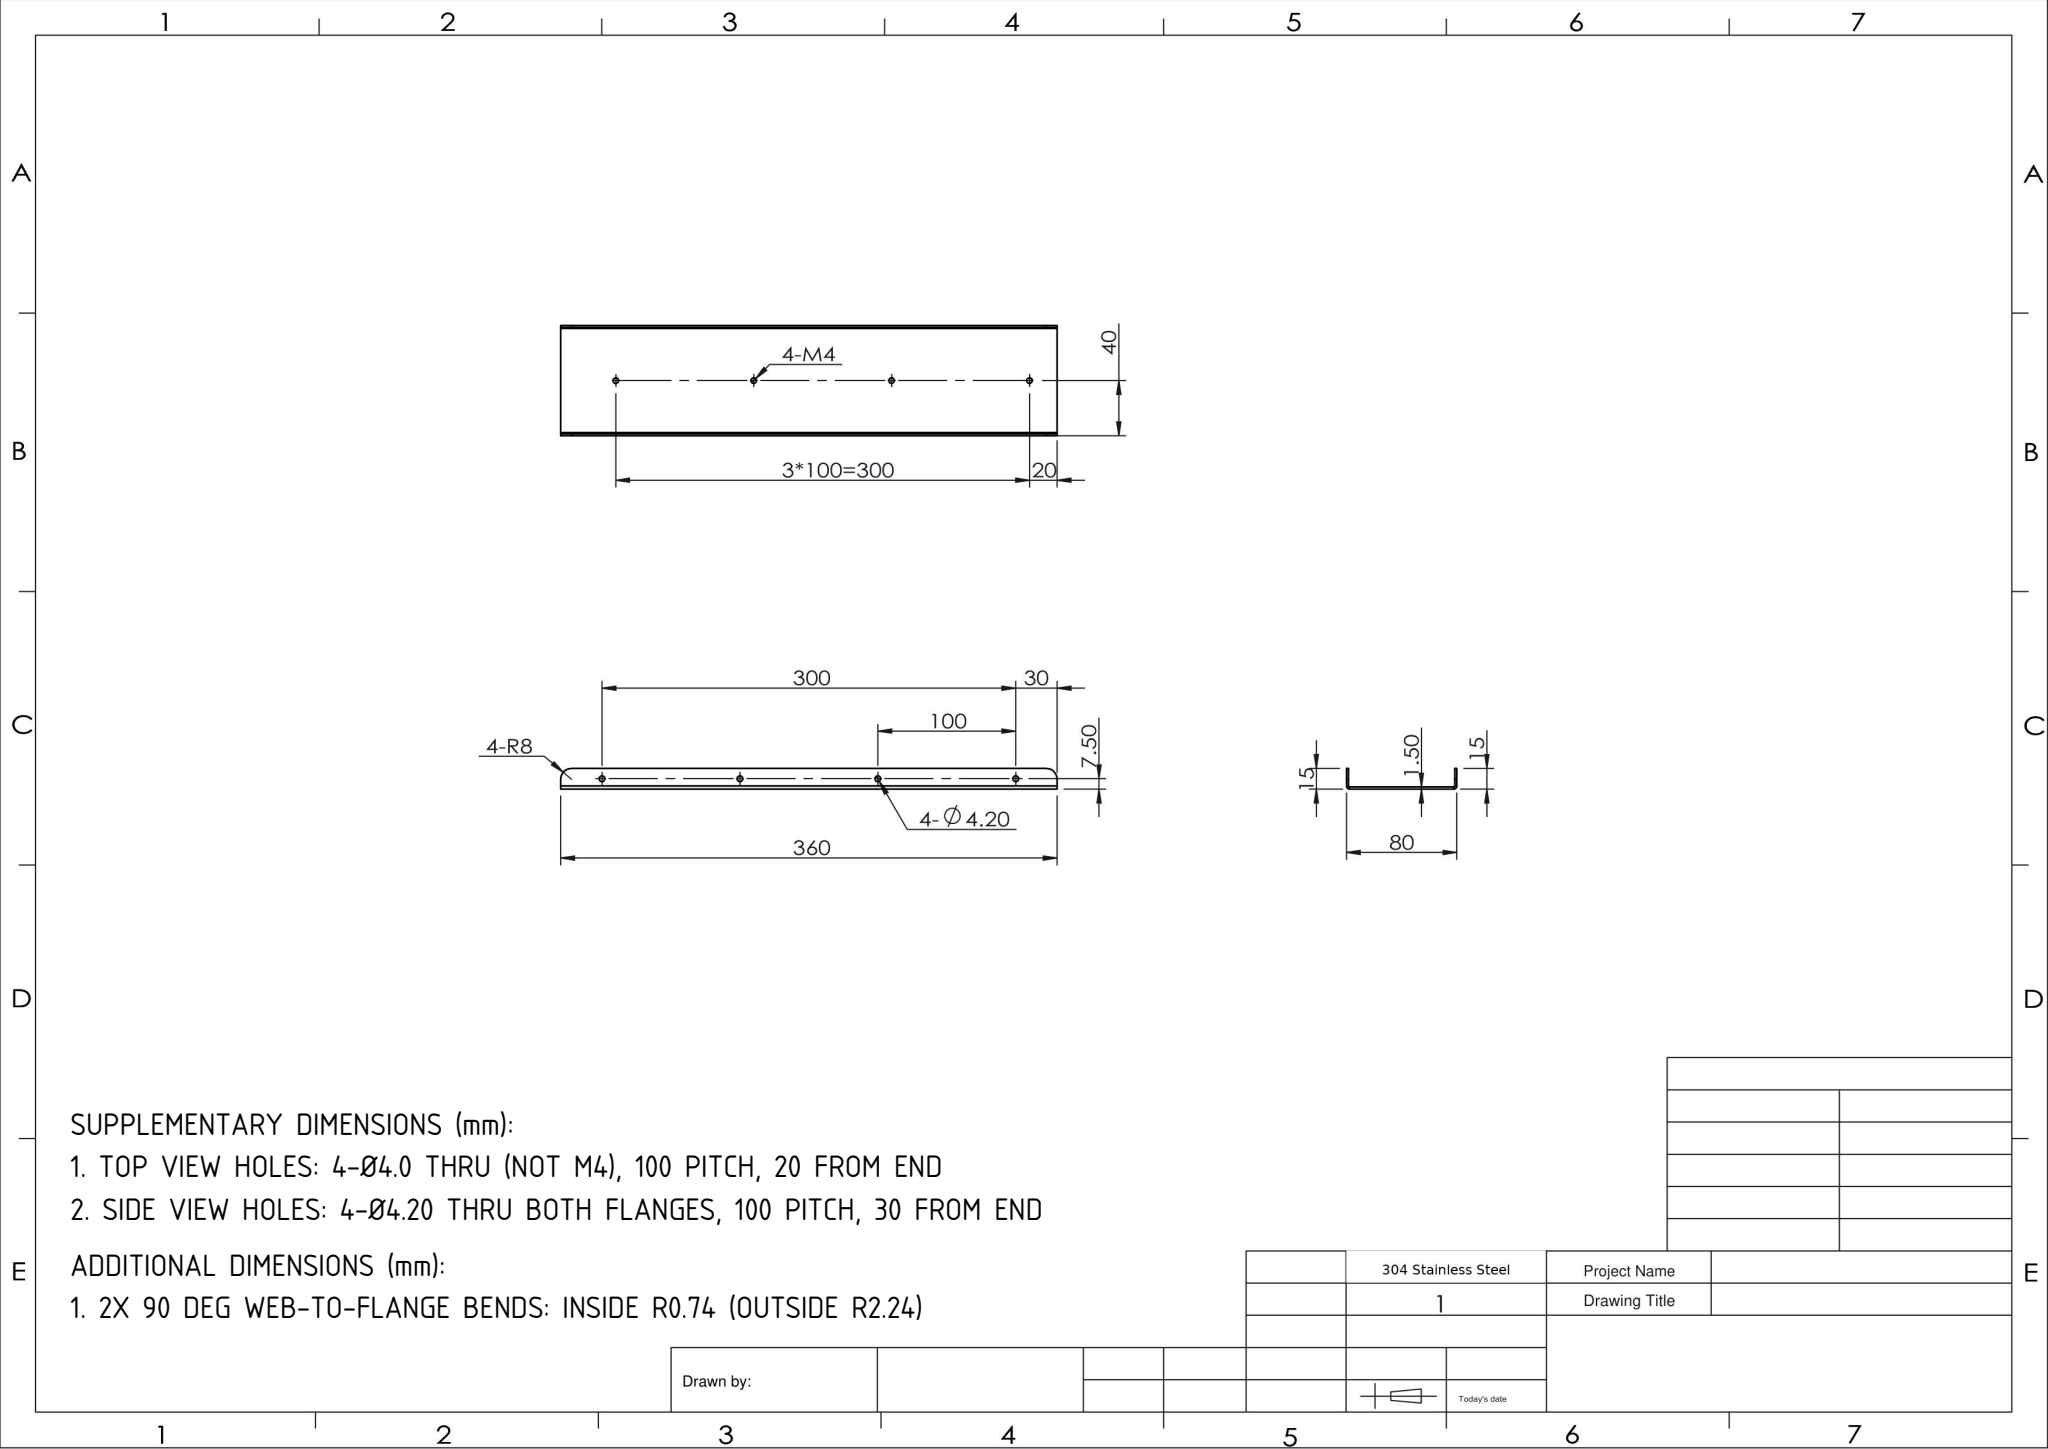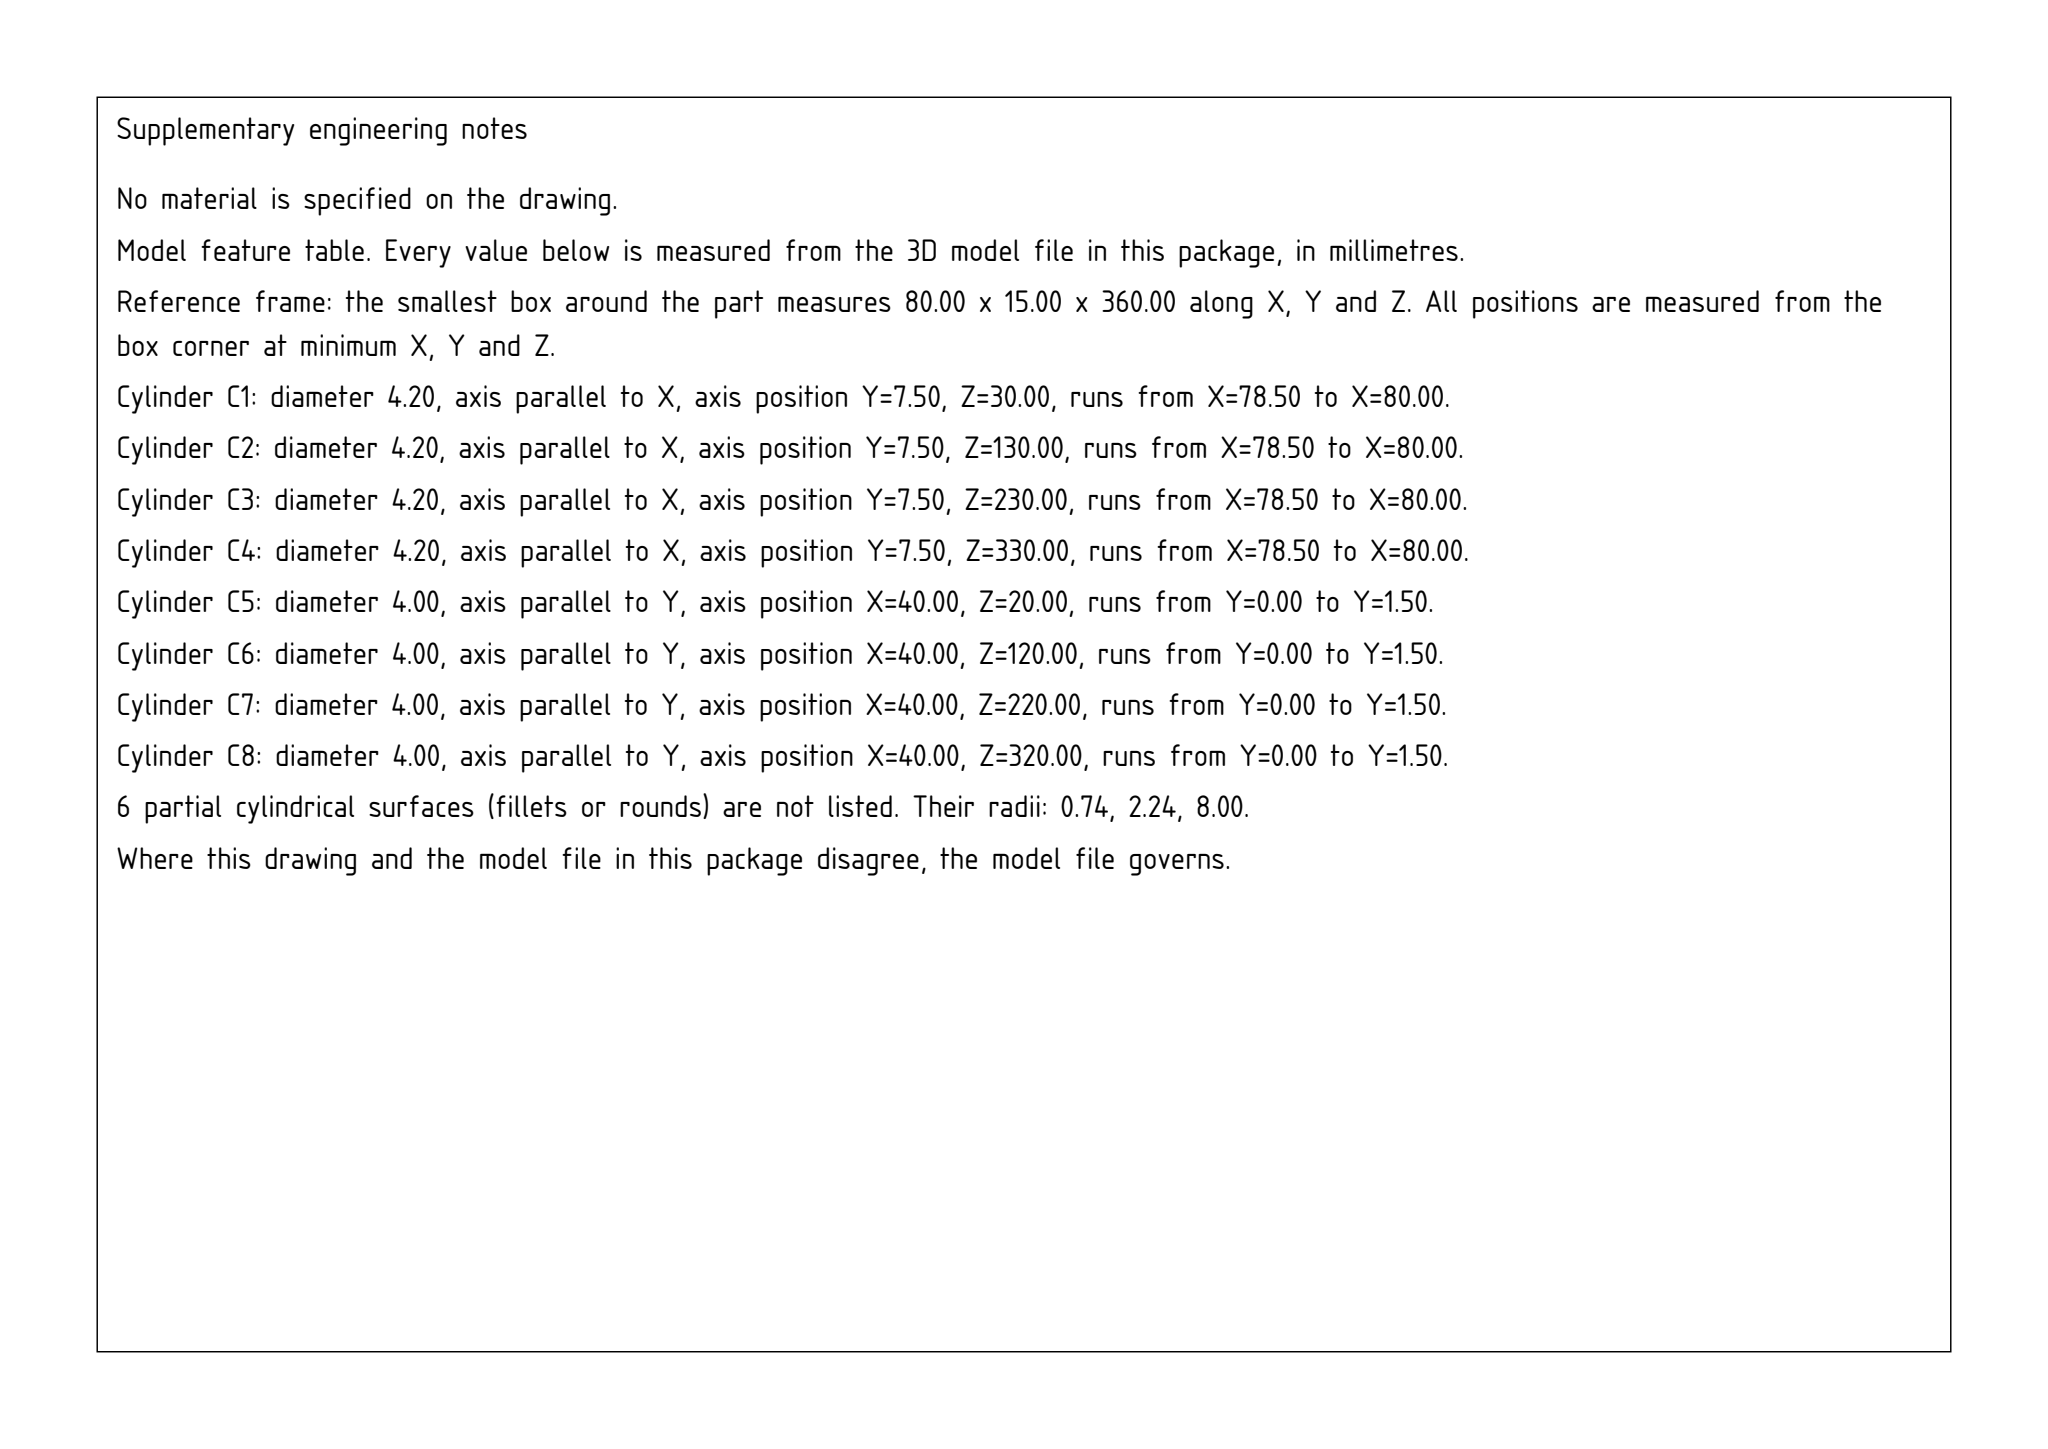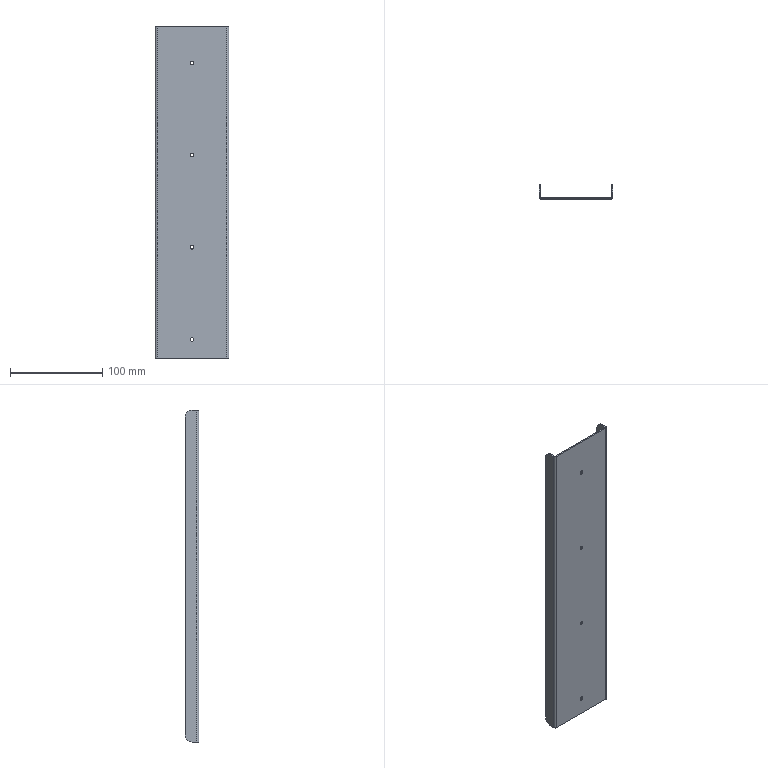Part | SolidWorks | mm | 1 solid | 42 faces | box 80 x 15 x 360 mm | volume 56850 mm3 | cylinder 24 | plane 18 | commonest cylinder face diameters 4 x8 4.2 x8 16 x4 4.473 x2 1.473 x2